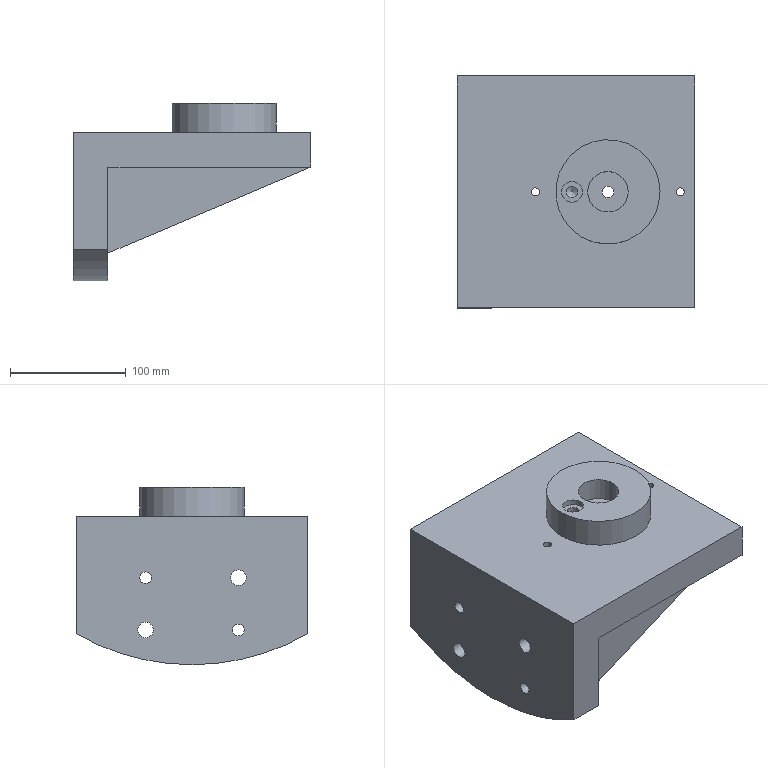Component | NX | ANGLE_IRON | 1 solid | 35 faces | volume 2010474 mm3 | plane 20 | cylinder 14 | cone 1 | commonest cylinder face diameters 10 x4 13.5 x2 20 x2 6.985 x2 400 x1 90 x1 35 x1 18 x1